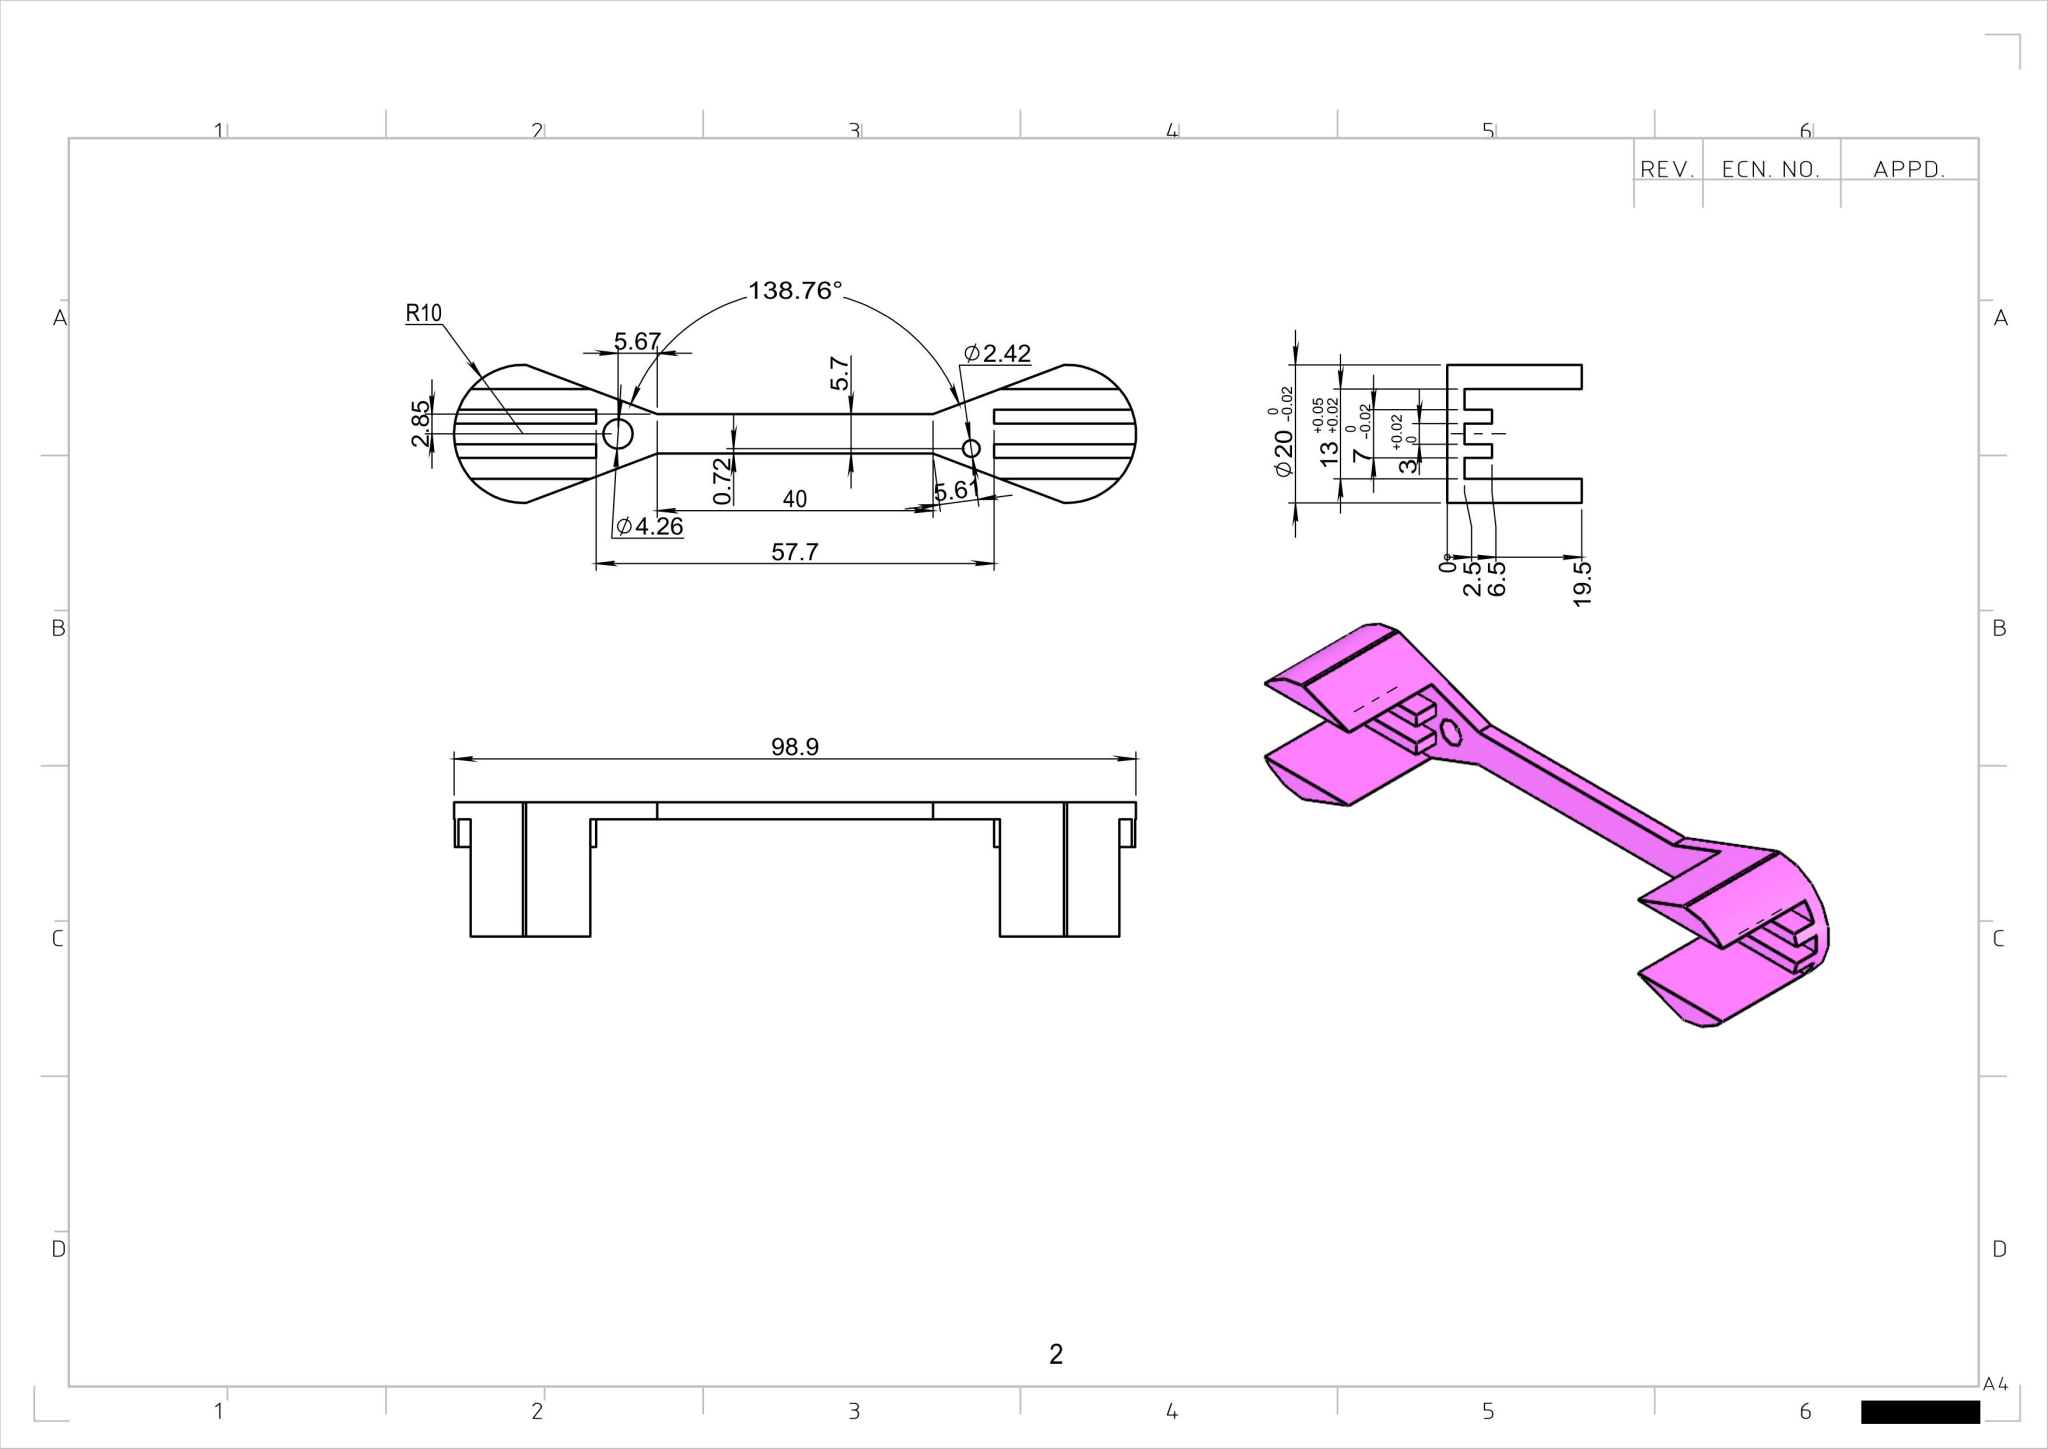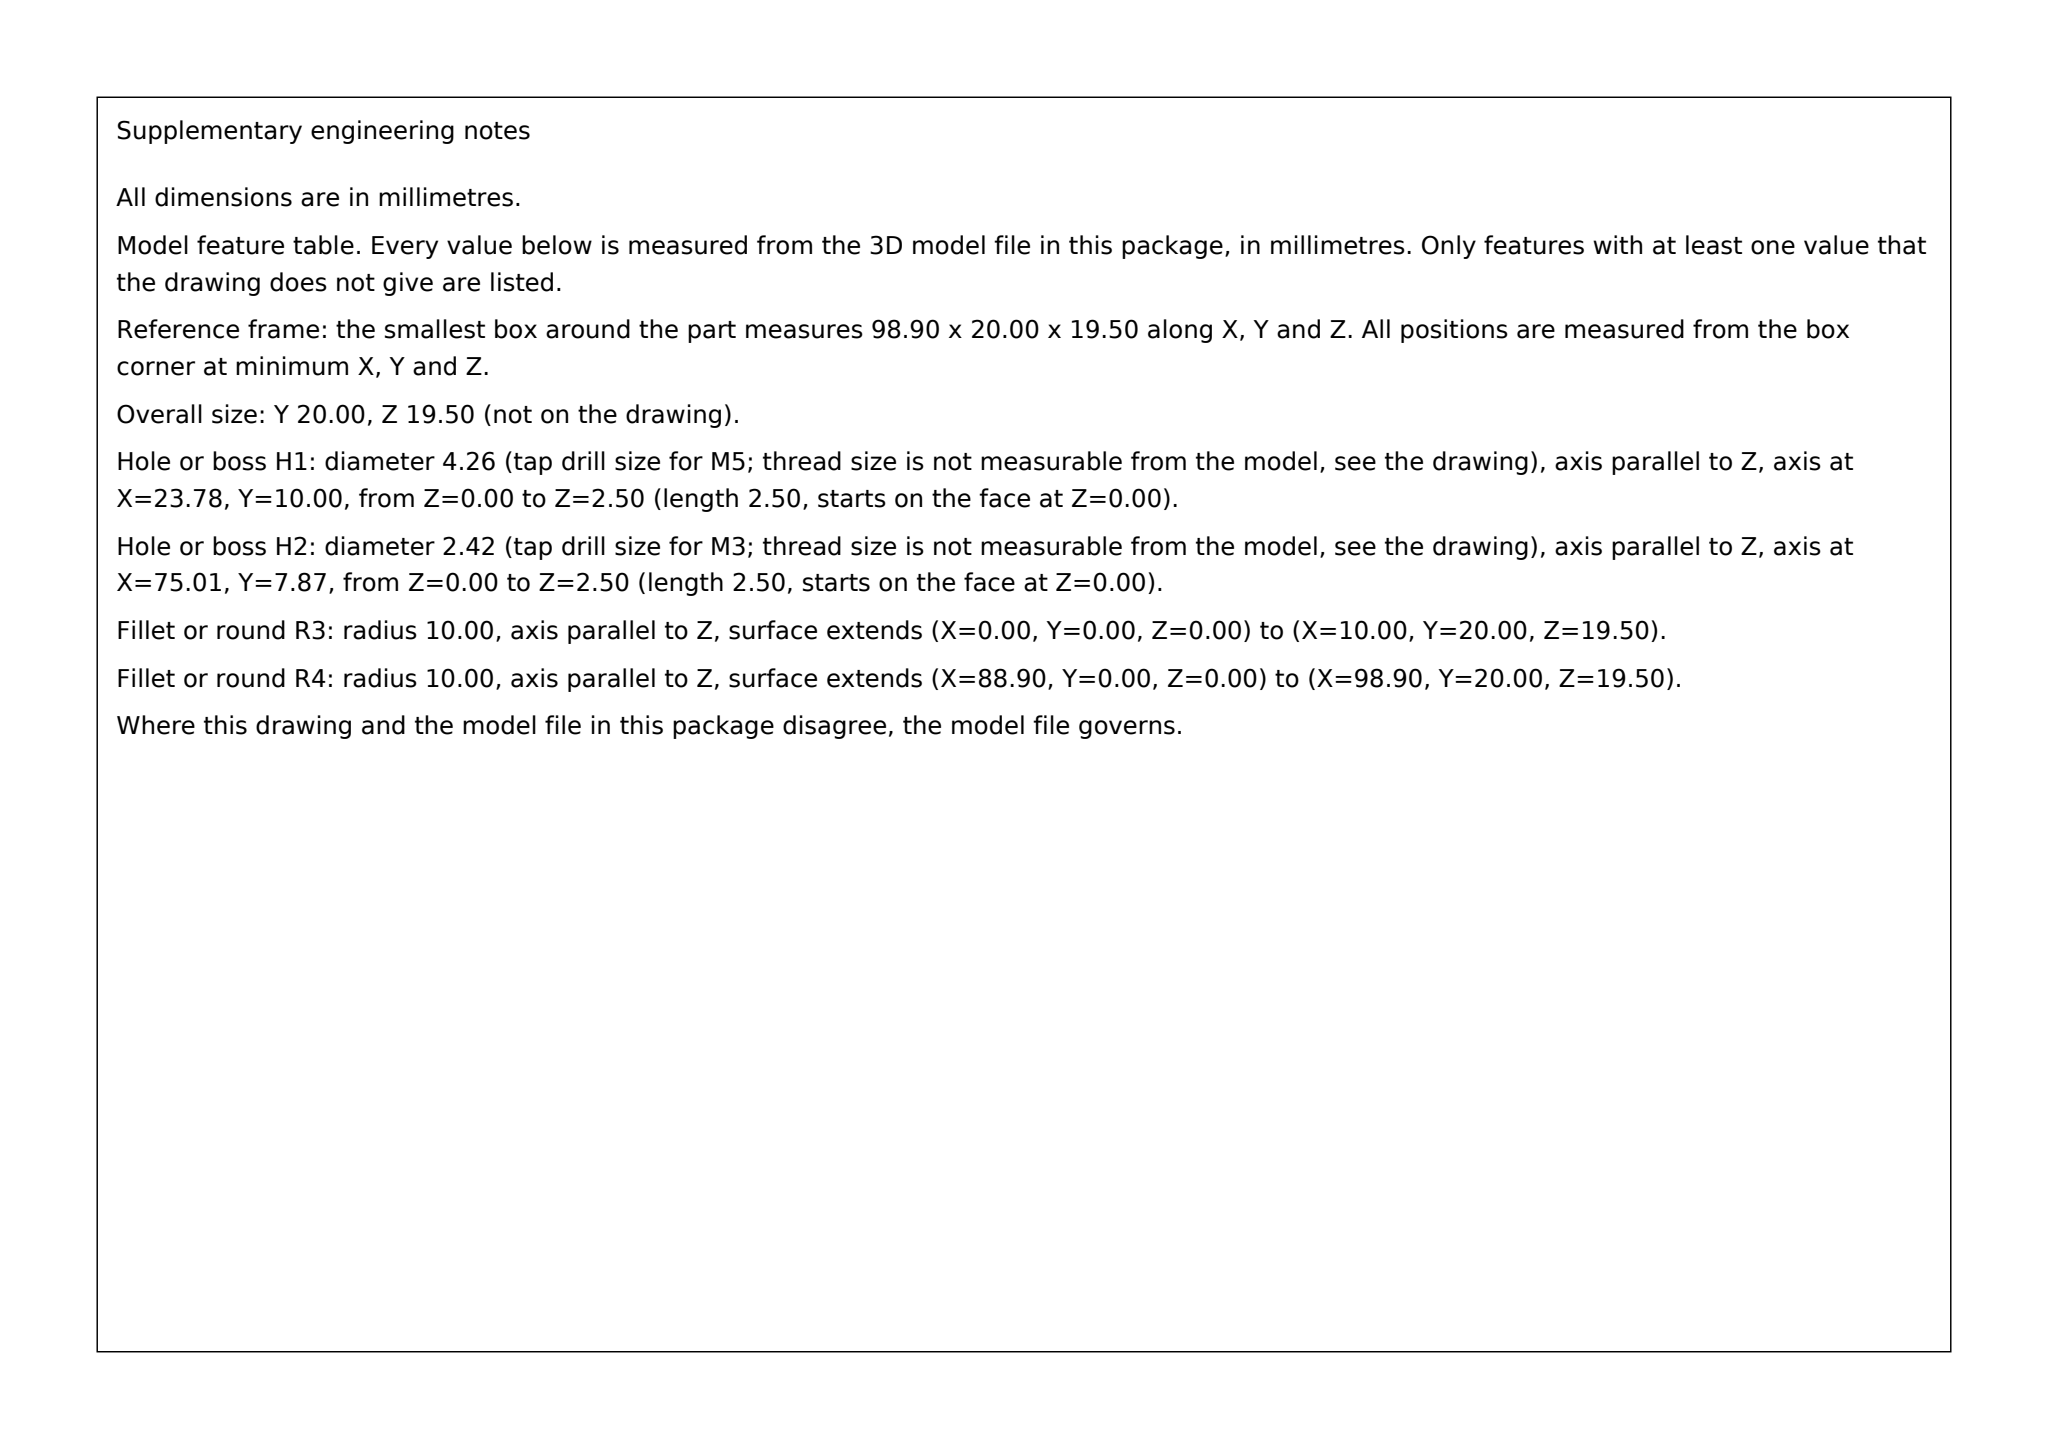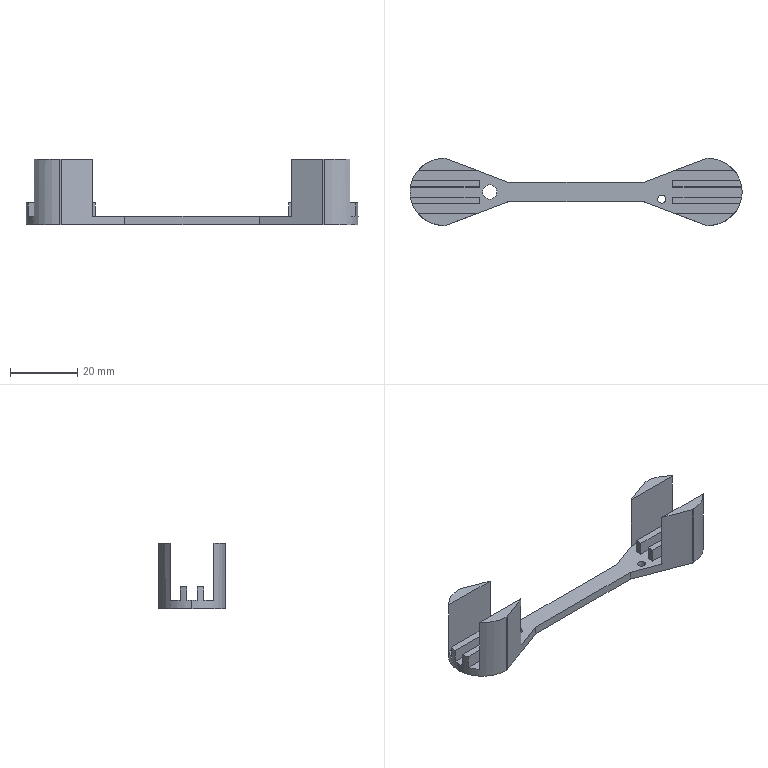Part | SolidWorks | mm | 1 solid | 43 faces | box 98.9 x 20 x 19.5 mm | volume 5692 mm3 | plane 36 | cylinder 7 | commonest cylinder face diameters 20 x3 4.258 x2 2.423 x2
build123d program:
from build123d import *

# Parameters (mm, degrees)
BOSS_EXTRUDE1_DEPTH     = 19.5
CUT_EXTRUDE1_DEPTH      = 55.088
CUT_EXTRUDE2_DEPTH      = 55.088
CUT_EXTRUDE2_DEPTH_BACK = 55.088
SKETCH4_W               = 57.7
SKETCH4_H               = 24.691
CUT_EXTRUDE3_DEPTH      = 54.238
SKETCH5_R               = 2.129
SKETCH5_R_2             = 1.212
CUT_EXTRUDE4_DEPTH      = 80


with BuildPart() as part:
    # Sketch1 → Boss-Extrude1 (new body)
    with BuildSketch(Plane.XY):
        with BuildLine():
            Line((-39.45, 10), (39.45, 10))
            ThreePointArc((39.45, 10), (49.45, 0), (39.45, -10))
            Line((39.45, -10), (-39.45, -10))
            ThreePointArc((-39.45, -10), (-49.45, 0), (-39.45, 10))
        make_face()
    extrude(amount=BOSS_EXTRUDE1_DEPTH)

    # Sketch2 → Cut-Extrude1 (cut, through all)
    with BuildSketch(Plane.XY.offset(19.5)):
        Polygon((-39, 10), (-20, 2.85), (20, 2.85), (39, 10), align=None)
        Polygon((-39, -10), (39, -10), (20, -2.85), (-20, -2.85), align=None)
    extrude(amount=-CUT_EXTRUDE1_DEPTH, mode=Mode.SUBTRACT)

    # Sketch3 → Cut-Extrude2 (cut, two sides: drawn at the far end of the back side and taken through both)
    with BuildSketch(Plane(origin=(0, 0, 0), x_dir=(0, 0, -1), z_dir=(1, 0, 0)).offset(-CUT_EXTRUDE2_DEPTH_BACK)):
        Polygon((-36.5, -6.5), (-2.5, -6.5), (-2.5, -3.5), (-6.5, -3.5), (-6.5, -1.5), (-2.5, -1.5), (-2.5, 1.5), (-6.5, 1.5), (-6.5, 3.5), (-2.5, 3.5), (-2.5, 6.5), (-36.5, 6.5), align=None)
    extrude(amount=CUT_EXTRUDE2_DEPTH + CUT_EXTRUDE2_DEPTH_BACK, mode=Mode.SUBTRACT)

    # Sketch4 → Cut-Extrude3 (cut, through all)
    with BuildSketch(Plane.XY.offset(2.5)):
        Rectangle(SKETCH4_W, SKETCH4_H)
    extrude(amount=CUT_EXTRUDE3_DEPTH, mode=Mode.SUBTRACT)

    # Sketch5 → Cut-Extrude4 (cut)
    with BuildSketch(Plane.XY.offset(2.5)):
        with Locations((-25.671, 0)):
            Circle(SKETCH5_R)
        with Locations((25.561, -2.129)):
            Circle(SKETCH5_R_2)
    extrude(amount=-CUT_EXTRUDE4_DEPTH, mode=Mode.SUBTRACT)


solid = part.part